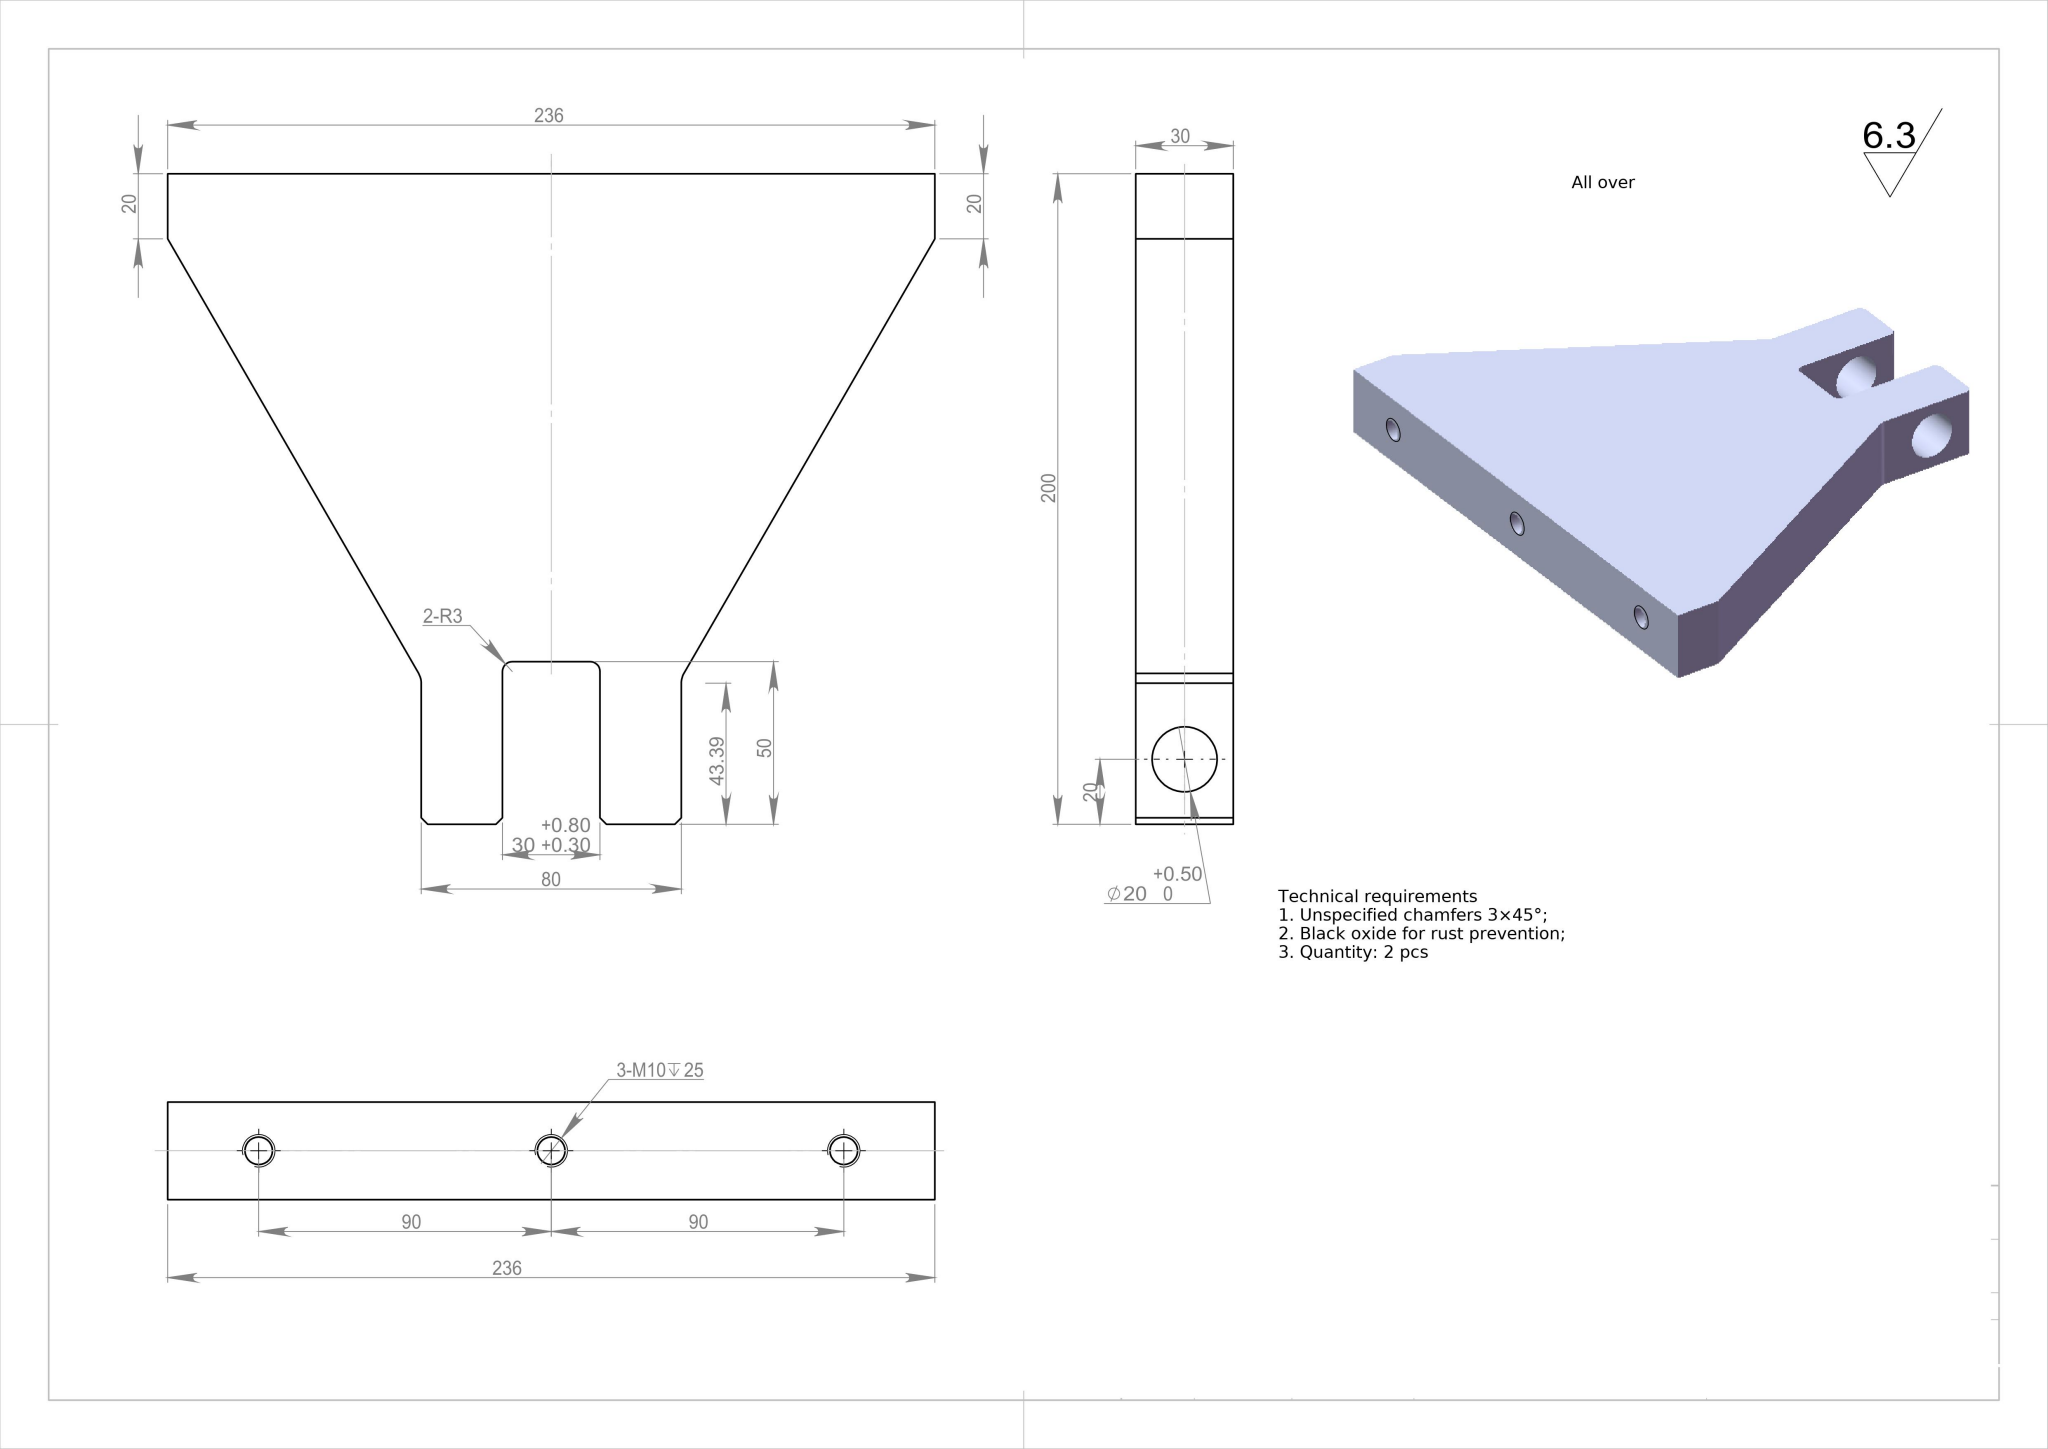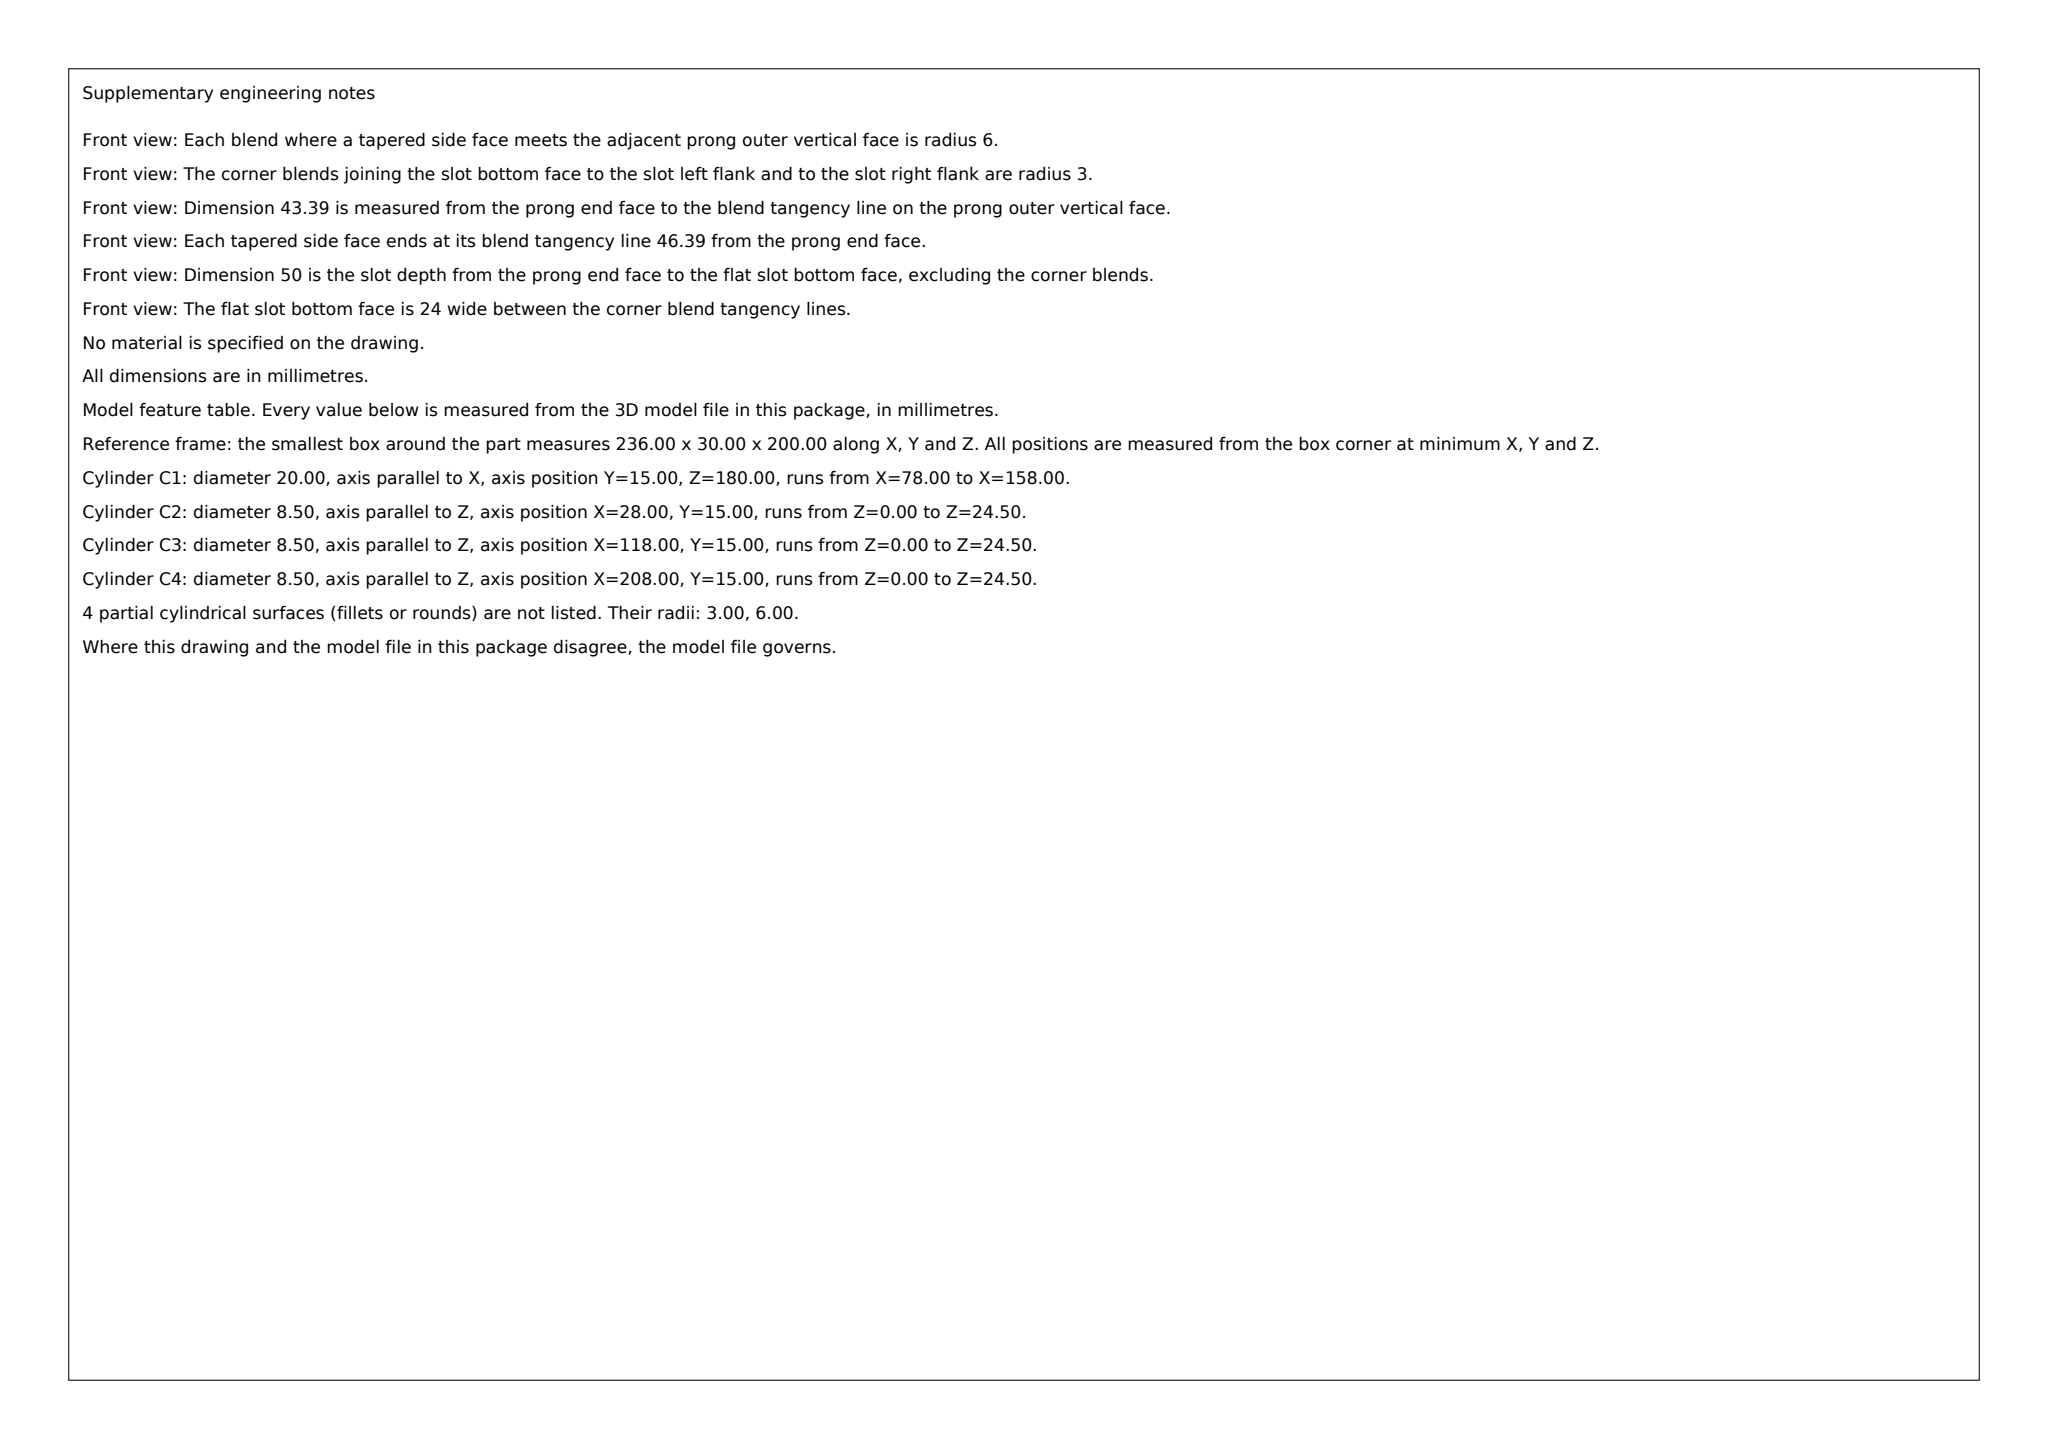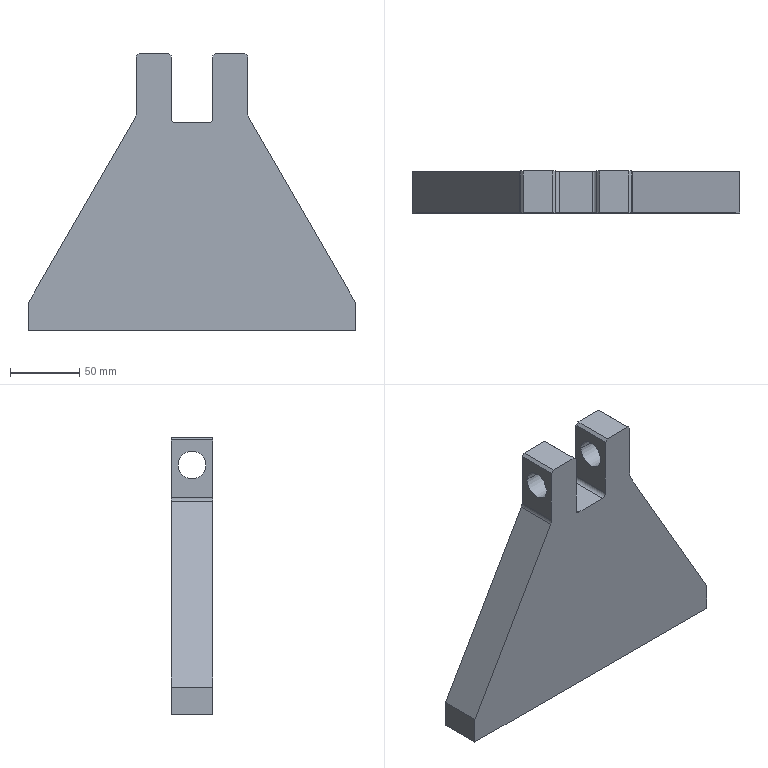Part | SolidWorks | mm | 1 solid | 38 faces | box 236 x 30 x 200 mm | volume 824366 mm3 | plane 18 | cylinder 14 | cone 6 | commonest cylinder face diameters 8.5 x6 20 x4 6 x2 12 x2
Drawing notes:
2X TAPERED SIDE FACES, SYMMETRIC ABOUT CENTRELINE: EACH RUNS FROM OUTER END FACE (X=0 AND X=236) AT 20 FROM MOUNTING (M10) FACE TO THE 80 WIDE CLEVIS FACES (X=78 AND X=158) AT 43.39 FROM CLEVIS END FACE; ≈25.6° TO CENTRELINE, TANGENT TO R6 BLENDS | from the solid: axis_planes x=0, x=78, x=158, x=236 and z=150/z=200; dia12 (R6) cylinders at z=156.61 (=200-43.39)
2X R6 BLEND RADIUS (Ø12 FULL ROUND, AXIS PARALLEL TO 30 THICKNESS) WHERE EACH TAPERED SIDE FACE MEETS THE VERTICAL OUTER FACE OF THE CLEVIS PRONG; CENTRES AT X=72 AND X=164 FROM LEFT END FACE, 43.39 FROM CLEVIS END FACE, THROUGH 30 THICKNESS | from the solid: cylinders [12.0,"y",[72.0,null,156.61],30.0] and [12.0,"y",[164.0,null,156.61],30.0]
CLEVIS: 2 PRONGS EACH 25 THICK (X=78 TO 103 AND X=133 TO 158) WITH 30 +0.80/+0.30 SLOT BETWEEN, SLOT BOTTOM 50 FROM CLEVIS END FACE; Ø20 +0.50/0 PIN HOLE THROUGH BOTH PRONGS, AXIS 20 FROM CLEVIS END FACE AND 15 FROM EACH 30 WIDE FACE | from the solid: axis_planes x=78,103,133,158 and z=150; cylinders [20.0,"x",[null,15.0,180.0],25.0,4]
build123d program:
from build123d import *

# Parameters (mm, degrees)
SKETCH1_W                                         = 236
SKETCH1_H                                         = 285
BOSS_EXTRUDE1_DEPTH                               = 20
SKETCH2_W                                         = 236
SKETCH2_H                                         = 30
BOSS_EXTRUDE2_DEPTH                               = 200
SKETCH3_W                                         = 30
SKETCH3_H                                         = 50
CUT_EXTRUDE1_DEPTH                                = 379.879
CHAMFER1_SIZE                                     = 2
FILLET1_R                                         = 3
SKETCH4_R                                         = 10
CUT_EXTRUDE2_DEPTH                                = 353.707
CUT_EXTRUDE3_DEPTH                                = 379.879
FILLET2_R                                         = 6
CHAMFER2_SIZE                                     = 2
HOLE_SIZE_ACCORDING_TO_TYPE_OF_HEXAGO_D           = 15.5
HOLE_SIZE_ACCORDING_TO_TYPE_OF_HEXAGO_DEPTH       = 22.25
HOLE_SIZE_ACCORDING_TO_TYPE_OF_HEXAGO_CBORE_D     = 24
HOLE_SIZE_ACCORDING_TO_TYPE_OF_HEXAGO_CBORE_DEPTH = 16
HOLE_SIZE_ACCORDING_TO_TYPE_OF_HEXAGO_TIP         = 4.657
SKETCH10_W                                        = 236
SKETCH10_H                                        = 20
CUT_EXTRUDE4_DEPTH                                = 379.879
M10_TAPPED_HOLE1_D                                = 8.5
M10_TAPPED_HOLE1_DEPTH                            = 24.5
M10_TAPPED_HOLE1_TIP                              = 2.554


with BuildPart() as part:
    # Sketch1 → Boss-Extrude1 (new body)
    with BuildSketch(Plane.XY):
        Rectangle(SKETCH1_W, SKETCH1_H)
    extrude(amount=BOSS_EXTRUDE1_DEPTH)

    # Sketch2 → Boss-Extrude2 (add)
    with BuildSketch(Plane.XY.offset(20)):
        with Locations((0, 127.5)):
            Rectangle(SKETCH2_W, SKETCH2_H)
    extrude(amount=BOSS_EXTRUDE2_DEPTH)

    # Sketch3 → Cut-Extrude1 (cut, through all)
    with BuildSketch(Plane(origin=(0, 142.5, 0), x_dir=(1, 0, 0), z_dir=(0, 1, 0))):
        with Locations((0, -195)):
            Rectangle(SKETCH3_W, SKETCH3_H)
    extrude(amount=-CUT_EXTRUDE1_DEPTH, mode=Mode.SUBTRACT)

    # Chamfer1
    chamfer1_edges = [part.edges().sort_by_distance(p)[0] for p in [
        (118, 127.5, 220),
        (-118, 127.5, 220),
        (118, -142.5, 10),
        (-118, -142.5, 10),
    ]]
    chamfer(chamfer1_edges, length=CHAMFER1_SIZE)

    # Fillet1
    fillet1_edges = [part.edges().sort_by_distance(p)[0] for p in [
        (-15, 127.5, 170),
        (15, 127.5, 170),
    ]]
    fillet(fillet1_edges, radius=FILLET1_R)

    # Sketch4 → Cut-Extrude2 (cut, through all)
    with BuildSketch(Plane(origin=(118, 0, 0), x_dir=(0, 0, -1), z_dir=(1, 0, 0))):
        with Locations(Location((-200, 127.5, 0), (0, 0, 90))):
            Circle(SKETCH4_R)
    extrude(amount=-CUT_EXTRUDE2_DEPTH, mode=Mode.SUBTRACT)

    # Sketch7 → Cut-Extrude3 (cut, through all)
    with BuildSketch(Plane(origin=(0, 142.5, 0), x_dir=(1, 0, 0), z_dir=(0, 1, 0))):
        Polygon((-118, -40), (-40, -175), (-40, -220), (-118, -220), align=None)
    cut_extrude3 = extrude(amount=-CUT_EXTRUDE3_DEPTH, mode=Mode.SUBTRACT)

    # Mirror2: Cut-Extrude3 across plane
    add(cut_extrude3.mirror(Plane(origin=(0, 0, 0), x_dir=(0, 0, 1), z_dir=(1, 0, 0))), mode=Mode.SUBTRACT)

    # Fillet2
    fillet2_edges = [part.edges().sort_by_distance(p)[0] for p in [
        (-40, 127.5, 175),
        (40, 127.5, 175),
    ]]
    fillet(fillet2_edges, radius=FILLET2_R)

    # Chamfer2
    chamfer2_edges = [part.edges().sort_by_distance(p)[0] for p in [
        (40, 127.5, 220),
        (15, 127.5, 220),
        (-15, 127.5, 220),
        (-40, 127.5, 220),
    ]]
    chamfer(chamfer2_edges, length=CHAMFER2_SIZE)

    # Hole Size _ according to_ type of Hexago
    with Locations(Plane(origin=(0, 0, 0), x_dir=(-1, 0, 0), z_dir=(0, 0, -1))):
        with Locations((-105, -129.5), (-105, -65.5), (105, -129.5), (105, -65.5)):
            CounterBoreHole(HOLE_SIZE_ACCORDING_TO_TYPE_OF_HEXAGO_D / 2, HOLE_SIZE_ACCORDING_TO_TYPE_OF_HEXAGO_CBORE_D / 2, HOLE_SIZE_ACCORDING_TO_TYPE_OF_HEXAGO_CBORE_DEPTH, depth=HOLE_SIZE_ACCORDING_TO_TYPE_OF_HEXAGO_DEPTH)
            with Locations((0, 0, -(HOLE_SIZE_ACCORDING_TO_TYPE_OF_HEXAGO_DEPTH + HOLE_SIZE_ACCORDING_TO_TYPE_OF_HEXAGO_TIP / 2))):  # 118° drill point
                Cone(0, HOLE_SIZE_ACCORDING_TO_TYPE_OF_HEXAGO_D / 2, HOLE_SIZE_ACCORDING_TO_TYPE_OF_HEXAGO_TIP, mode=Mode.SUBTRACT)

    # Sketch10 → Cut-Extrude4 (cut, through all)
    with BuildSketch(Plane.XZ.offset(142.5)):
        with Locations((0, 10)):
            Rectangle(SKETCH10_W, SKETCH10_H)
    extrude(amount=-CUT_EXTRUDE4_DEPTH, mode=Mode.SUBTRACT)

    # M10 Tapped Hole1
    with Locations(Plane(origin=(0, 0, 20), x_dir=(-1, 0, 0), z_dir=(0, 0, -1))):
        with Locations((0, 127.5), (-90, 127.5), (90, 127.5)):
            Hole(M10_TAPPED_HOLE1_D / 2, depth=M10_TAPPED_HOLE1_DEPTH)
            with Locations((0, 0, -(M10_TAPPED_HOLE1_DEPTH + M10_TAPPED_HOLE1_TIP / 2))):  # 118° drill point
                Cone(0, M10_TAPPED_HOLE1_D / 2, M10_TAPPED_HOLE1_TIP, mode=Mode.SUBTRACT)


solid = part.part